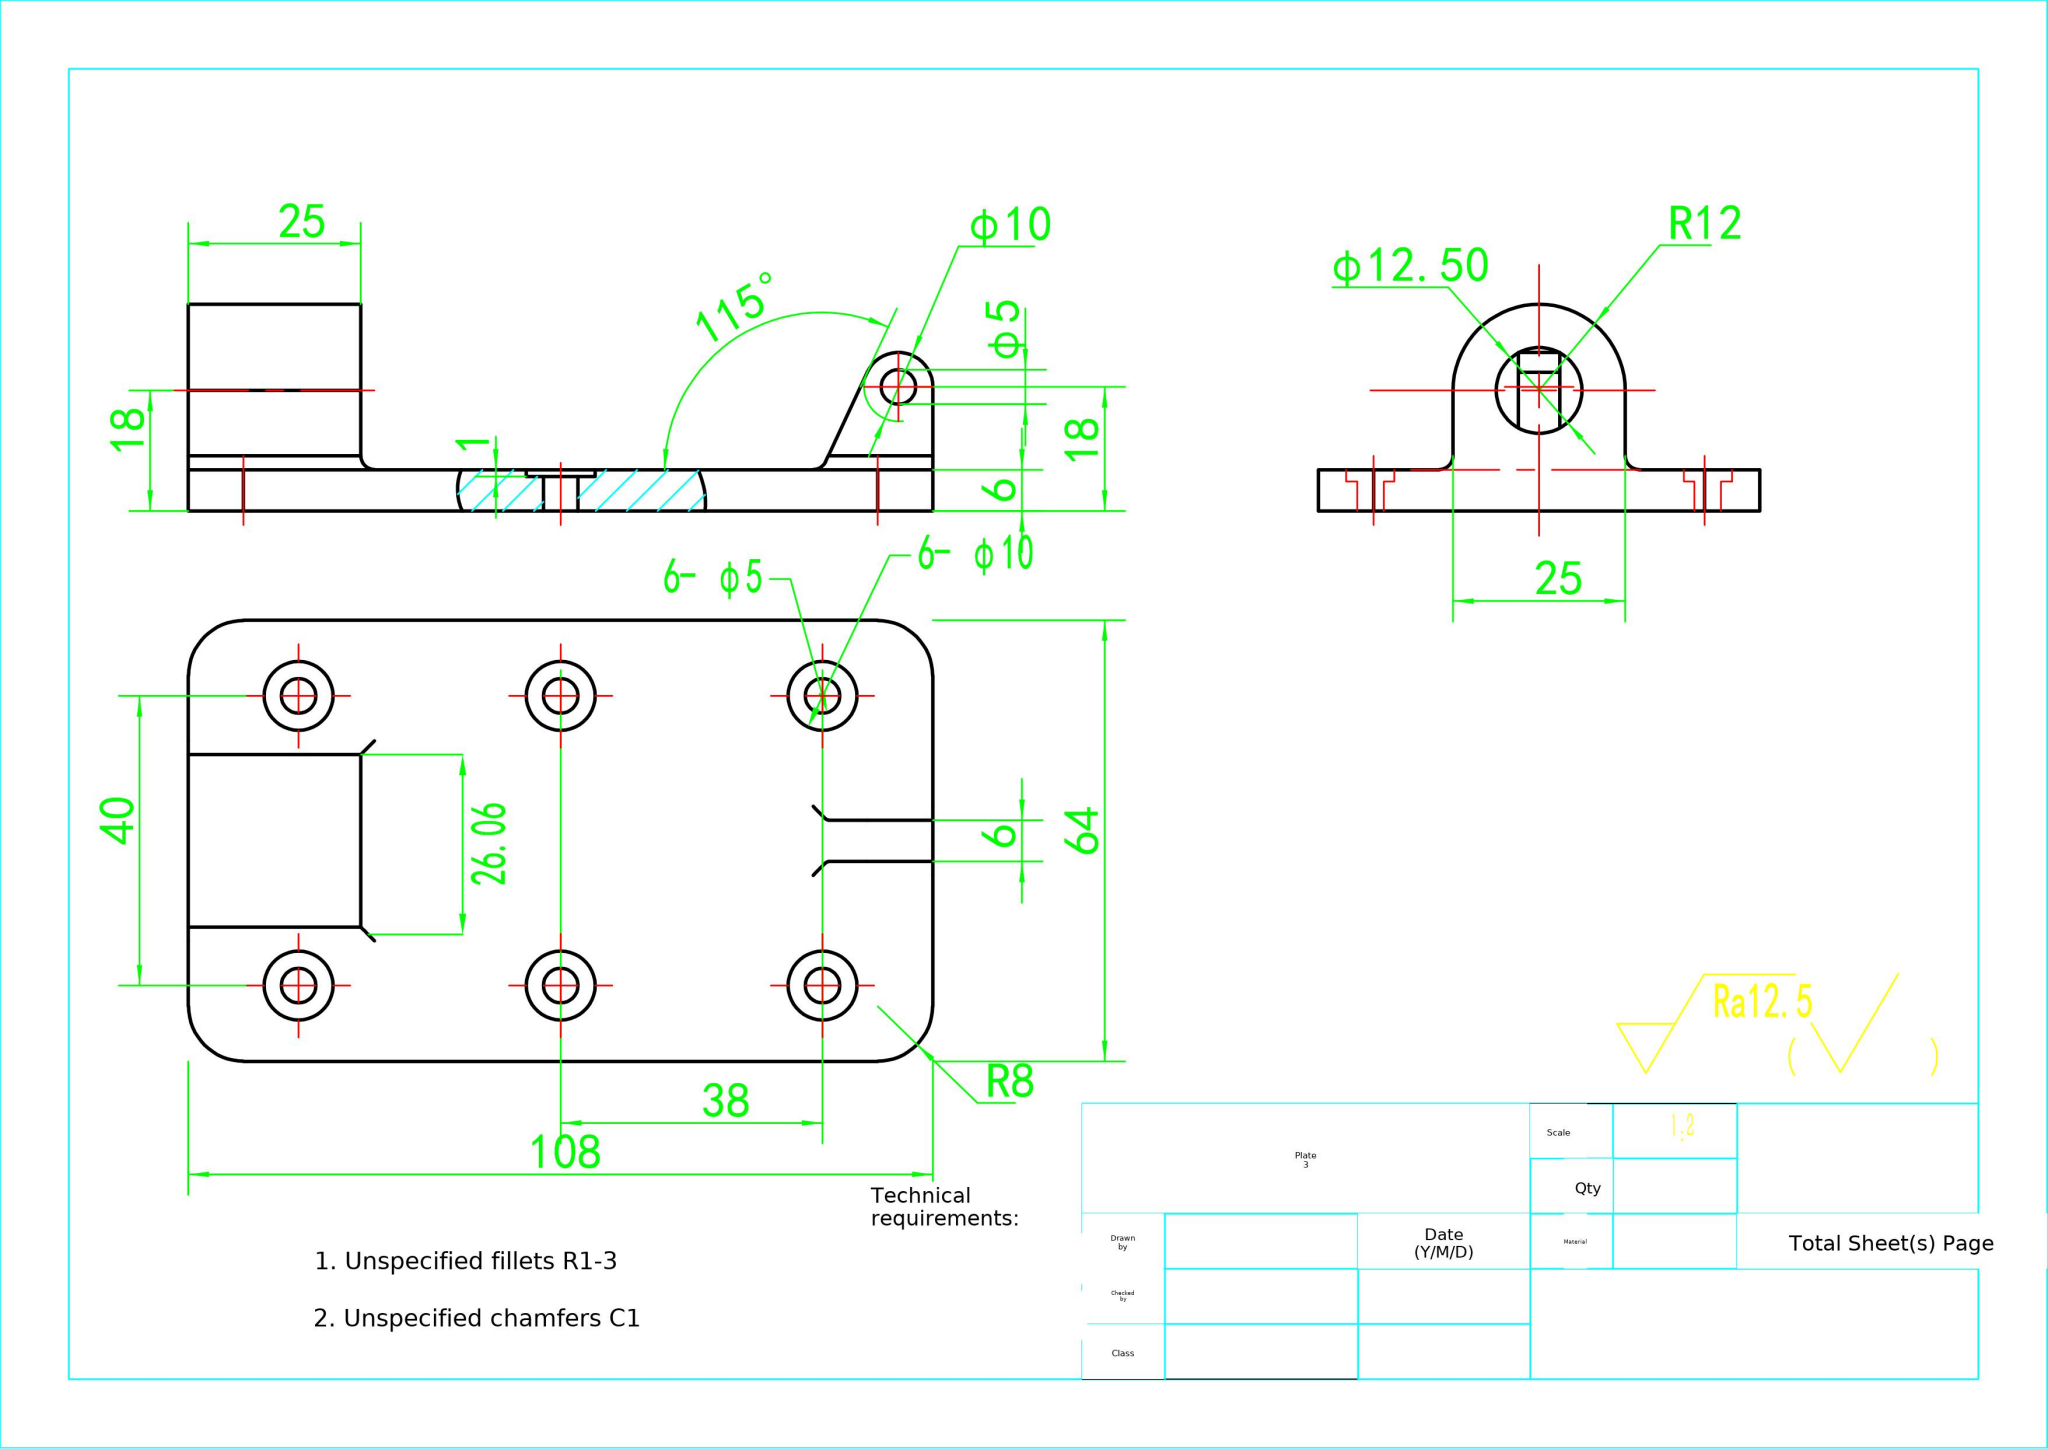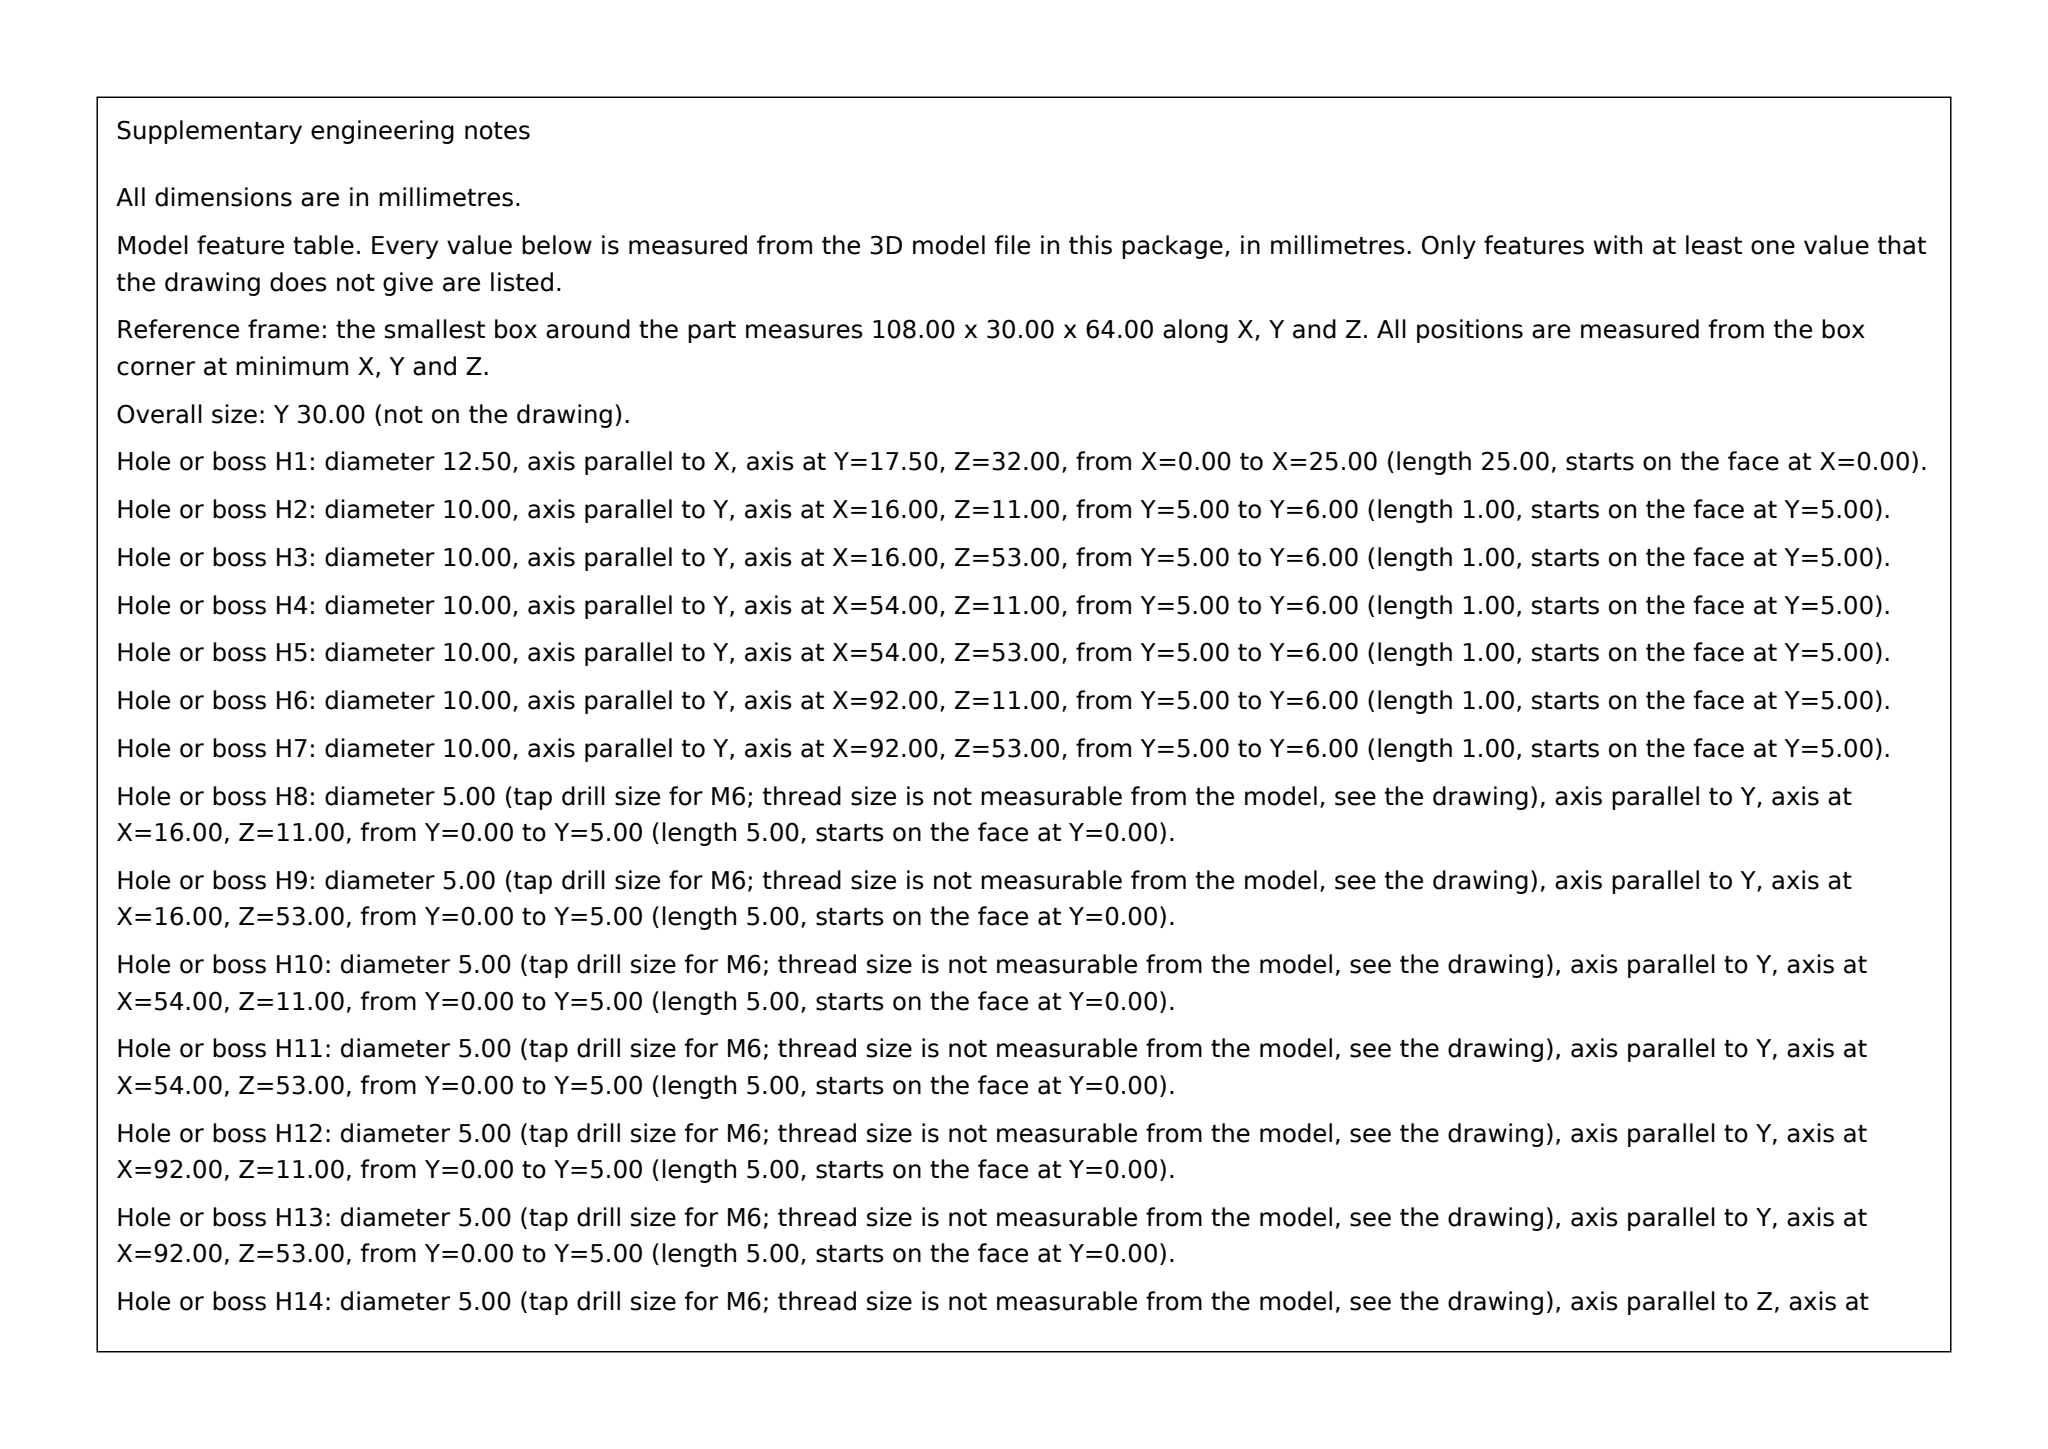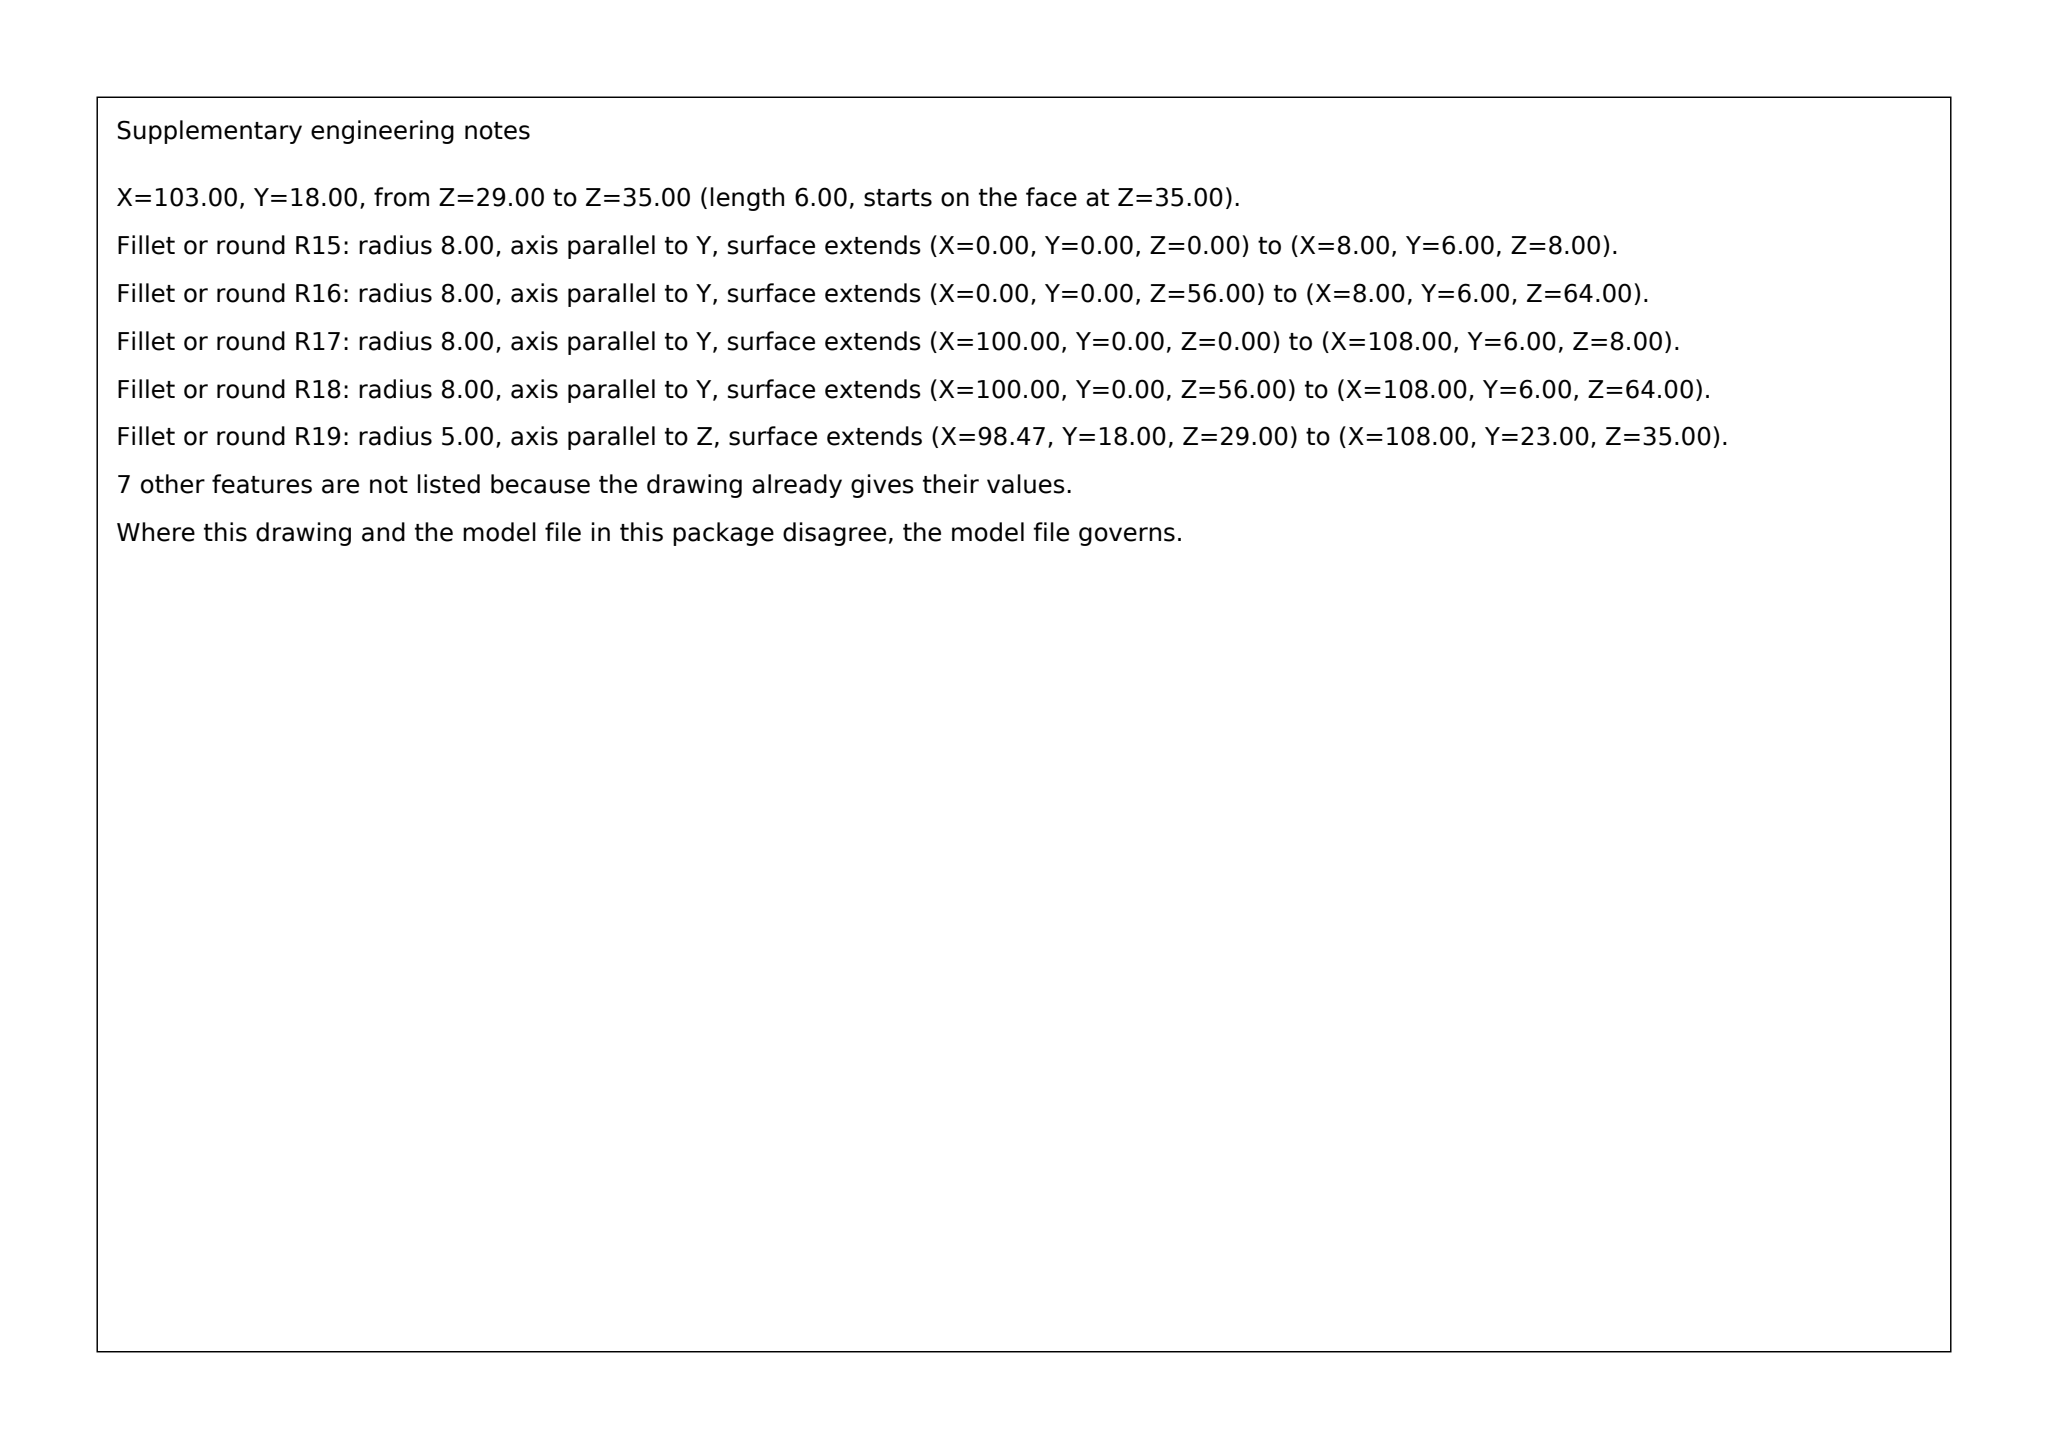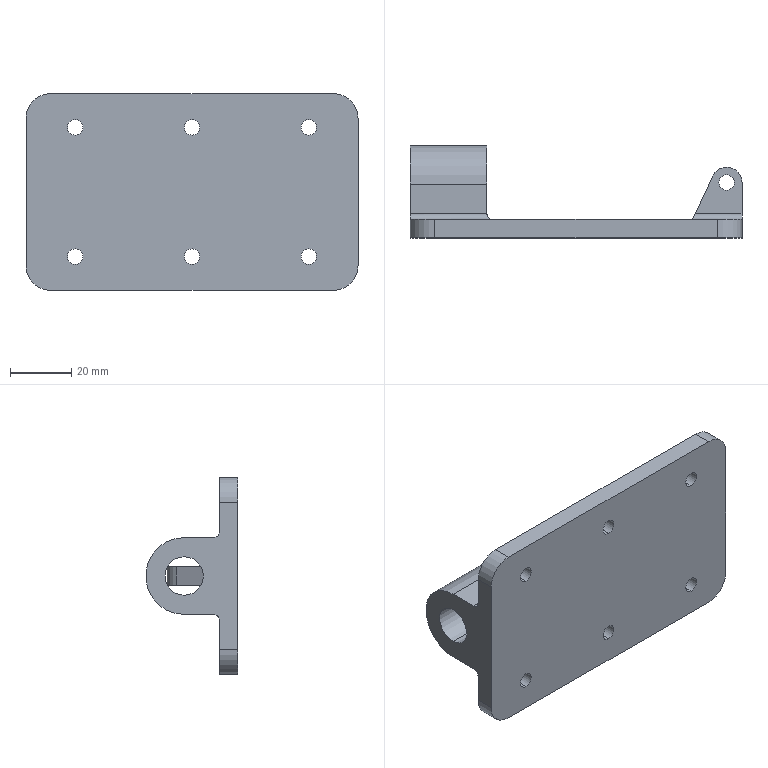Part | SolidWorks | mm | 1 solid | 58 faces | box 108 x 30 x 64 mm | volume 51512 mm3 | cylinder 40 | plane 18 | commonest cylinder face diameters 5 x14 10 x13 4 x6 16 x4 12.5 x2 25 x1
build123d program:
from build123d import *

# Parameters (mm, degrees)
BOSS_EXTRUDE1_DEPTH = 6
SKETCH2_W           = 25
SKETCH2_H           = 25
BOSS_EXTRUDE2_DEPTH = 24
CUT_EXTRUDE1_DEPTH  = 51
SKETCH4_R           = 6.25
CUT_EXTRUDE2_DEPTH  = 63
FILLET1_R           = 2
FILLET2_R           = 2
SKETCH5_R           = 2.5
BOSS_EXTRUDE3_DEPTH = 3
FILLET3_R           = 2
HOLE1_D             = 5
HOLE1_DEPTH         = 100
HOLE1_CBORE_D       = 10
HOLE1_CBORE_DEPTH   = 1


with BuildPart() as part:
    # Sketch1 → Boss-Extrude1 (new body)
    with BuildSketch(Plane(origin=(0, 0, 0), x_dir=(1, 0, 0), z_dir=(0, 1, 0))):
        with BuildLine():
            Line((-46, -32), (46, -32))
            ThreePointArc((46, -32), (51.657, -29.657), (54, -24))
            Line((54, -24), (54, 24))
            ThreePointArc((54, 24), (51.657, 29.657), (46, 32))
            Line((46, 32), (-46, 32))
            ThreePointArc((-46, 32), (-51.657, 29.657), (-54, 24))
            Line((-54, 24), (-54, -24))
            ThreePointArc((-54, -24), (-51.657, -29.657), (-46, -32))
        make_face()
    extrude(amount=BOSS_EXTRUDE1_DEPTH)

    # Sketch2 → Boss-Extrude2 (add)
    with BuildSketch(Plane(origin=(0, 6, 0), x_dir=(1, 0, 0), z_dir=(0, 1, 0))):
        with Locations((-41.5, 0)):
            Rectangle(SKETCH2_W, SKETCH2_H)
    extrude(amount=BOSS_EXTRUDE2_DEPTH)

    # Sketch3 → Cut-Extrude1 (cut)
    with BuildSketch(Plane(origin=(-29, 0, 0), x_dir=(0, 0, -1), z_dir=(1, 0, 0))):
        with BuildLine():
            Line((-12.5, 30), (-12.5, 17.5))
            ThreePointArc((-12.5, 17.5), (-8.839, 26.339), (0, 30))
            Line((0, 30), (-12.5, 30))
        make_face()
        with BuildLine():
            ThreePointArc((0, 30), (8.839, 26.339), (12.5, 17.5))
            Line((12.5, 17.5), (12.5, 30))
            Line((12.5, 30), (0, 30))
        make_face()
    extrude(amount=-CUT_EXTRUDE1_DEPTH, mode=Mode.SUBTRACT)

    # Sketch4 → Cut-Extrude2 (cut)
    with BuildSketch(Plane(origin=(-29, 0, 0), x_dir=(0, 0, -1), z_dir=(1, 0, 0))):
        with Locations((0, 17.5)):
            Circle(SKETCH4_R)
    extrude(amount=-CUT_EXTRUDE2_DEPTH, mode=Mode.SUBTRACT)

    # Fillet1
    fillet1_edges = [part.edges().sort_by_distance(p)[0] for p in [
        (-41.5, 6, 12.5),
    ]]
    fillet(fillet1_edges, radius=FILLET1_R)

    # Fillet2
    fillet2_edges = [part.edges().sort_by_distance(p)[0] for p in [
        (-41.5, 6, -12.5),
        (-29, 6, 1),
    ]]
    fillet(fillet2_edges, radius=FILLET2_R)

    # Sketch5 → Boss-Extrude3 (add, symmetric)
    with BuildSketch(Plane.XY):
        with BuildLine():
            Line((54, 18), (54, 6))
            Line((54, 6), (37.887, 6))
            Line((37.887, 6), (43.483, 18))
            Line((43.483, 18), (44.468, 20.113))
            ThreePointArc((44.468, 20.113), (50.082, 22.881), (54, 18))
        make_face()
        with Locations((49, 18)):
            Circle(SKETCH5_R, mode=Mode.SUBTRACT)
    extrude(amount=BOSS_EXTRUDE3_DEPTH, both=True)

    # Fillet3
    fillet3_edges = [part.edges().sort_by_distance(p)[0] for p in [
        (45.944, 6, 3),
        (45.944, 6, -3),
        (37.887, 6, 0),
    ]]
    fillet(fillet3_edges, radius=FILLET3_R)

    # Hole1
    with Locations(Plane(origin=(0, 6, -21), x_dir=(0, 0, 1), z_dir=(0, 1, 0))):
        with Locations((0, 0), (0, 38), (0, -38)):
            hole1 = CounterBoreHole(HOLE1_D / 2, HOLE1_CBORE_D / 2, HOLE1_CBORE_DEPTH, depth=HOLE1_DEPTH)

    # Mirror1: Hole1 across plane
    add(hole1.mirror(Plane.XY), mode=Mode.SUBTRACT)


solid = part.part